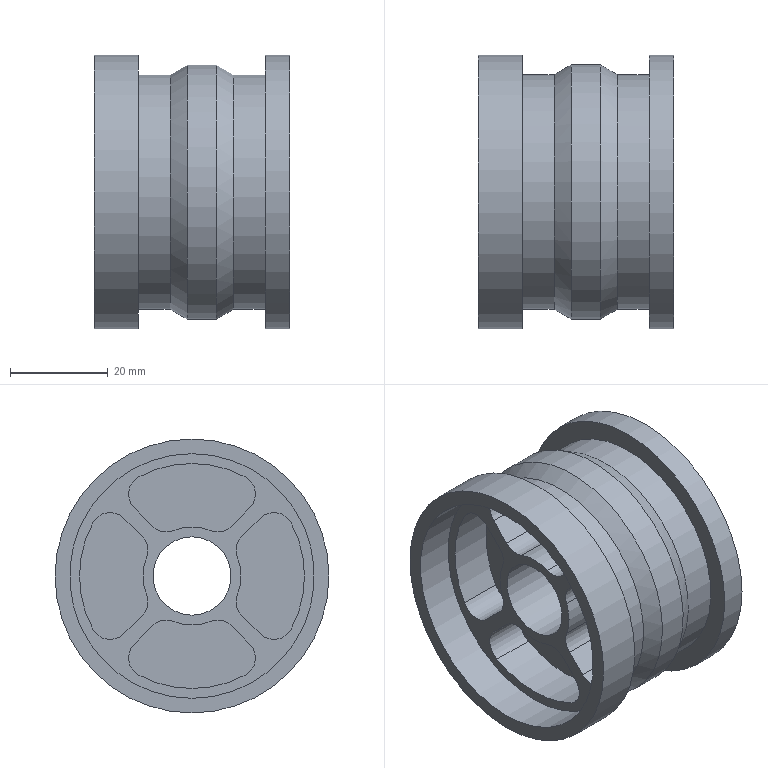Component | NX | WHEEL_2 | 1 solid | 54 faces | volume 32605 mm3 | cylinder 33 | plane 19 | cone 2 | commonest cylinder face diameters 8 x16 20 x4 46 x4 56 x2 48 x2 50 x1 16 x1 22 x1